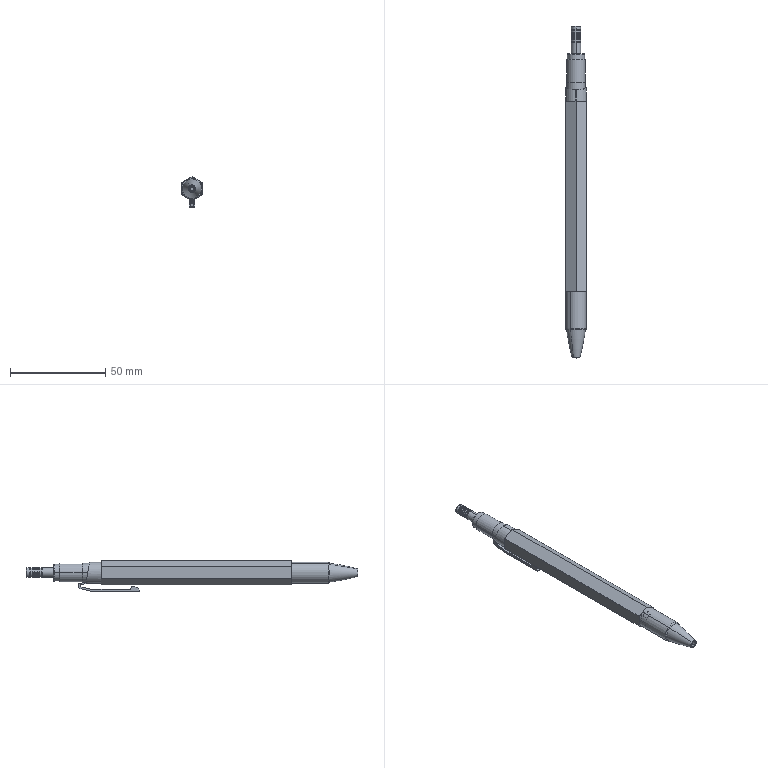Assembly | SolidWorks | mm | 7 component files | 7 solids | 288 faces | box 11 x 174.5 x 16.17 mm | volume 4237 mm3 | cylinder 160 | plane 77 | torus 20 | spline 19 | cone 12 | commonest cylinder face diameters 10 x73 5 x18 4.5 x12 3 x8 4 x8 2 x6 9 x6 8 x6
Bill of materials:
CompressionSpringSpringConstant0.2-0.5D5L10 | 1 |  | Cylindrical helical coil of round-section wire with constant diameter and open pitch along the body. The end coils are closely spaced or touching, and both wire ends are cut square. Its shape resembles a helical compression spring.
PenBody | 1 |  | Long, straight hollow shaft with a hexagonal middle section and stepped round journals at both ends. One end has a narrow band with fine ridges next to the hex shoulder.
PenHolder | 1 |  | Formed thin strip part: a short open cylindrical band (split ring with a narrow axial gap) joined to a long, flat, angled arm that leaves the band tangentially. The arm has a jog/bend near the band and ends in a forked tip with two rounded lobes.
PenRefillTube | 1 |  | Long, slender, straight tube of uniform circular cross-section with plain square-cut ends.
PenTail | 1 |  | Hollow, axisymmetric tubular part: a thin central neck between two larger cylindrical end collars. One collar has an open plain end; the other has a chamfered or tapered outer end.
PenTailCap | 1 |  | Headed cylindrical pin or plug: a large flat circular flange at one end, a cylindrical shank, and a series of evenly spaced circumferential grooves near the shank's rounded far end. The flange face has a circular recess.
PenTip | 1 |  | Hollow, axisymmetric nozzle-like body: a straight cylindrical section followed by a conical taper ending in a small open tip, with a small step at the joint between the cylinder and the cone.
Mates:
1. concentric | PenTail-1 face at (-56.698, 35.736, -29.961) dir (0, -1, 0) r 2.5 | PenRefillTube-1 face at (-56.698, 40.236, -29.961) dir (0, -1, 0) r 1.5
2. concentric | PenBody-1 face at (-56.698, -100.264, -29.961) dir (0, -1, 0) r 4 | PenTail-1 face at (-56.698, 35.736, -29.961) dir (0, -1, 0) r 2.5
3. concentric | PenHolder-1 face at (-56.698, 25.736, -29.961) dir (0, -1, 0) r 5 | PenBody-1 face at (-56.698, 17.736, -29.961) dir (0, -1, 0) r 5
4. coincident | PenHolder-1 face at (-56.698, 17.736, -29.961) dir (0, -1, 0) | PenBody-1 face at (-56.698, 17.736, -29.961) dir (0, 1, 0)
5. concentric | PenBody-1 face at (-56.698, 17.736, -29.961) dir (0, -1, 0) r 4.75 | PenTailCap-1 face at (-56.698, 40.236, -29.961) dir (0, -1, 0) r 4
6. coincident | PenBody-1 face at (-56.698, 42.236, -29.961) dir (0, -1, 0) | PenTailCap-1 face at (-56.698, 42.236, -33.961) dir (0, 1, 0)
7. coincident | PenTail-1 face at (-56.698, 56.736, -31.961) dir (0, 1, 0) | PenTailCap-1 edge at (-56.698, 56.736, -29.961) dir (0, -1, 0) r 2
8. concentric | PenBody-1 face at (-56.698, -100.264, -29.961) dir (0, -1, 0) r 4 | PenTip-1 face at (-56.698, -82.264, -29.961) dir (0, 1, 0) r 5.5
9. coincident | PenBody-1 face at (-56.698, -82.264, -29.961) dir (0, -1, 0) | PenTip-1 face at (-56.698, -82.264, -29.961) dir (0, 1, 0)
10. tangent | PenTail-1 face at (-56.698, 40.986, -29.961) dir (1, 0, 0) | PenRefillTube-1 face at (-56.698, 40.236, -29.961) dir (0, 1, 0)
11. coincident | PenBody-1 plane at (-56.698, -100.264, -29.961) dir (0, 0, 1) | CompressionSpringSpringConstant0.2-0.5D5L10-1 plane at (-56.698, -109.255, -29.961) dir (0, 0, 1)
12. coincident | PenRefillTube-1 plane at (-56.698, -104.764, -29.961) dir (-1, 0, 0) | CompressionSpringSpringConstant0.2-0.5D5L10-1 plane at (-56.698, -109.255, -29.961) dir (1, 0, 0)